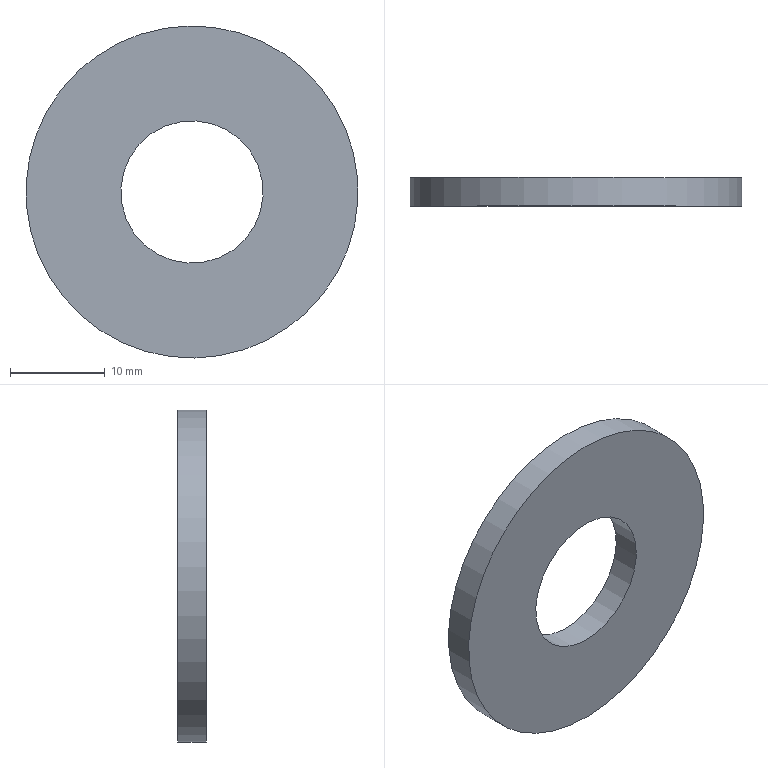Component | NX | RETAINING_RING | 1 solid | 4 faces | box 35 x 3 x 35 mm | volume 2356 mm3 | cylinder 2 | plane 2 | commonest cylinder face diameters 35 x1 15 x1
STEP:
#1=CARTESIAN_POINT('',(0.,0.,0.));
#2=DIRECTION('',(0.,0.,1.));
#3=DIRECTION('',(1.,0.,0.));
#4=AXIS2_PLACEMENT_3D('',#1,#2,#3);
#5=CARTESIAN_POINT('',(646.363,-282.302,-1469.318));
#6=VERTEX_POINT('',#5);
#7=CARTESIAN_POINT('',(630.189,-282.302,-1476.));
#8=DIRECTION('',(0.,-1.,0.));
#9=DIRECTION('',(0.9242,0.,0.3818));
#10=AXIS2_PLACEMENT_3D('',#7,#8,#9);
#11=CIRCLE('',#10,17.5);
#12=CARTESIAN_POINT('',(630.189,-282.302,-1476.));
#13=DIRECTION('',(0.,1.,0.));
#14=DIRECTION('',(-0.9242,0.,-0.3818));
#15=AXIS2_PLACEMENT_3D('',#12,#13,#14);
#16=CYLINDRICAL_SURFACE('',#15,17.5);
#17=CARTESIAN_POINT('',(9.425,0.));
#18=DIRECTION('',(-1.,0.));
#19=VECTOR('',#18,1.);
#20=LINE('',#17,#19);
#21=(GEOMETRIC_REPRESENTATION_CONTEXT(2)PARAMETRIC_REPRESENTATION_CONTEXT()REPRESENTATION_CONTEXT('',''));
#22=DEFINITIONAL_REPRESENTATION('',(#20),#21);
#23=PCURVE('',#16,#22);
#24=CARTESIAN_POINT('',(630.189,-282.302,-1476.));
#25=DIRECTION('',(0.,-1.,0.));
#26=DIRECTION('',(0.9242,0.,0.3818));
#27=AXIS2_PLACEMENT_3D('',#24,#25,#26);
#28=PLANE('',#27);
#29=CARTESIAN_POINT('',(0.,0.));
#30=DIRECTION('',(1.,0.));
#31=AXIS2_PLACEMENT_2D('',#29,#30);
#32=CIRCLE('',#31,17.5);
#33=(GEOMETRIC_REPRESENTATION_CONTEXT(2)PARAMETRIC_REPRESENTATION_CONTEXT()REPRESENTATION_CONTEXT('',''));
#34=DEFINITIONAL_REPRESENTATION('',(#32),#33);
#35=PCURVE('',#28,#34);
#36=SURFACE_CURVE('',#11,(#23,#35),.PCURVE_S1.);
#37=EDGE_CURVE('',#6,#6,#36,.T.);
#38=ORIENTED_EDGE('',*,*,#37,.F.);
#39=CARTESIAN_POINT('',(646.363,-279.302,-1469.318));
#40=VERTEX_POINT('',#39);
#41=CARTESIAN_POINT('',(646.363,-282.302,-1469.318));
#42=CARTESIAN_POINT('',(646.363,-279.302,-1469.318));
#43=B_SPLINE_CURVE_WITH_KNOTS('',1,(#41,#42),.UNSPECIFIED.,.F.,.F.,(2,2),(0.,3.),.PIECEWISE_BEZIER_KNOTS.);
#44=CARTESIAN_POINT('',(9.425,0.));
#45=DIRECTION('',(0.,1.));
#46=VECTOR('',#45,1.);
#47=LINE('',#44,#46);
#48=(GEOMETRIC_REPRESENTATION_CONTEXT(2)PARAMETRIC_REPRESENTATION_CONTEXT()REPRESENTATION_CONTEXT('',''));
#49=DEFINITIONAL_REPRESENTATION('',(#47),#48);
#50=PCURVE('',#16,#49);
#51=CARTESIAN_POINT('',(3.142,0.));
#52=DIRECTION('',(0.,1.));
#53=VECTOR('',#52,1.);
#54=LINE('',#51,#53);
#55=(GEOMETRIC_REPRESENTATION_CONTEXT(2)PARAMETRIC_REPRESENTATION_CONTEXT()REPRESENTATION_CONTEXT('',''));
#56=DEFINITIONAL_REPRESENTATION('',(#54),#55);
#57=PCURVE('',#16,#56);
#58=SEAM_CURVE('',#43,(#50,#57),.PCURVE_S1.);
#59=EDGE_CURVE('',#6,#40,#58,.T.);
#60=ORIENTED_EDGE('',*,*,#59,.T.);
#61=CARTESIAN_POINT('',(630.189,-279.302,-1476.));
#62=DIRECTION('',(0.,-1.,0.));
#63=DIRECTION('',(0.9242,0.,0.3818));
#64=AXIS2_PLACEMENT_3D('',#61,#62,#63);
#65=CIRCLE('',#64,17.5);
#66=CARTESIAN_POINT('',(9.425,3.));
#67=DIRECTION('',(-1.,0.));
#68=VECTOR('',#67,1.);
#69=LINE('',#66,#68);
#70=(GEOMETRIC_REPRESENTATION_CONTEXT(2)PARAMETRIC_REPRESENTATION_CONTEXT()REPRESENTATION_CONTEXT('',''));
#71=DEFINITIONAL_REPRESENTATION('',(#69),#70);
#72=PCURVE('',#16,#71);
#73=CARTESIAN_POINT('',(630.189,-279.302,-1476.));
#74=DIRECTION('',(0.,-1.,0.));
#75=DIRECTION('',(0.9242,0.,0.3818));
#76=AXIS2_PLACEMENT_3D('',#73,#74,#75);
#77=PLANE('',#76);
#78=CARTESIAN_POINT('',(0.,0.));
#79=DIRECTION('',(1.,0.));
#80=AXIS2_PLACEMENT_2D('',#78,#79);
#81=CIRCLE('',#80,17.5);
#82=(GEOMETRIC_REPRESENTATION_CONTEXT(2)PARAMETRIC_REPRESENTATION_CONTEXT()REPRESENTATION_CONTEXT('',''));
#83=DEFINITIONAL_REPRESENTATION('',(#81),#82);
#84=PCURVE('',#77,#83);
#85=SURFACE_CURVE('',#65,(#72,#84),.PCURVE_S1.);
#86=EDGE_CURVE('',#40,#40,#85,.T.);
#87=ORIENTED_EDGE('',*,*,#86,.T.);
#88=ORIENTED_EDGE('',*,*,#59,.F.);
#89=EDGE_LOOP('',(#38,#60,#87,#88));
#90=FACE_BOUND('',#89,.T.);
#91=ADVANCED_FACE('',(#90),#16,.T.);
#92=CARTESIAN_POINT('',(637.121,-282.302,-1473.136));
#93=VERTEX_POINT('',#92);
#94=CARTESIAN_POINT('',(630.189,-282.302,-1476.));
#95=DIRECTION('',(0.,-1.,0.));
#96=DIRECTION('',(0.9242,0.,0.3818));
#97=AXIS2_PLACEMENT_3D('',#94,#95,#96);
#98=CIRCLE('',#97,7.5);
#99=CARTESIAN_POINT('',(630.189,-282.302,-1476.));
#100=DIRECTION('',(0.,1.,0.));
#101=DIRECTION('',(-0.9242,0.,-0.3818));
#102=AXIS2_PLACEMENT_3D('',#99,#100,#101);
#103=CYLINDRICAL_SURFACE('',#102,7.5);
#104=CARTESIAN_POINT('',(9.425,0.));
#105=DIRECTION('',(-1.,0.));
#106=VECTOR('',#105,1.);
#107=LINE('',#104,#106);
#108=(GEOMETRIC_REPRESENTATION_CONTEXT(2)PARAMETRIC_REPRESENTATION_CONTEXT()REPRESENTATION_CONTEXT('',''));
#109=DEFINITIONAL_REPRESENTATION('',(#107),#108);
#110=PCURVE('',#103,#109);
#111=CARTESIAN_POINT('',(0.,0.));
#112=DIRECTION('',(1.,0.));
#113=AXIS2_PLACEMENT_2D('',#111,#112);
#114=CIRCLE('',#113,7.5);
#115=(GEOMETRIC_REPRESENTATION_CONTEXT(2)PARAMETRIC_REPRESENTATION_CONTEXT()REPRESENTATION_CONTEXT('',''));
#116=DEFINITIONAL_REPRESENTATION('',(#114),#115);
#117=PCURVE('',#28,#116);
#118=SURFACE_CURVE('',#98,(#110,#117),.PCURVE_S1.);
#119=EDGE_CURVE('',#93,#93,#118,.T.);
#120=ORIENTED_EDGE('',*,*,#119,.F.);
#121=CARTESIAN_POINT('',(637.121,-279.302,-1473.136));
#122=VERTEX_POINT('',#121);
#123=CARTESIAN_POINT('',(637.121,-282.302,-1473.136));
#124=CARTESIAN_POINT('',(637.121,-279.302,-1473.136));
#125=B_SPLINE_CURVE_WITH_KNOTS('',1,(#123,#124),.UNSPECIFIED.,.F.,.F.,(2,2),(0.,3.),.PIECEWISE_BEZIER_KNOTS.);
#126=CARTESIAN_POINT('',(9.425,0.));
#127=DIRECTION('',(0.,1.));
#128=VECTOR('',#127,1.);
#129=LINE('',#126,#128);
#130=(GEOMETRIC_REPRESENTATION_CONTEXT(2)PARAMETRIC_REPRESENTATION_CONTEXT()REPRESENTATION_CONTEXT('',''));
#131=DEFINITIONAL_REPRESENTATION('',(#129),#130);
#132=PCURVE('',#103,#131);
#133=CARTESIAN_POINT('',(3.142,0.));
#134=DIRECTION('',(0.,1.));
#135=VECTOR('',#134,1.);
#136=LINE('',#133,#135);
#137=(GEOMETRIC_REPRESENTATION_CONTEXT(2)PARAMETRIC_REPRESENTATION_CONTEXT()REPRESENTATION_CONTEXT('',''));
#138=DEFINITIONAL_REPRESENTATION('',(#136),#137);
#139=PCURVE('',#103,#138);
#140=SEAM_CURVE('',#125,(#132,#139),.PCURVE_S1.);
#141=EDGE_CURVE('',#93,#122,#140,.T.);
#142=ORIENTED_EDGE('',*,*,#141,.T.);
#143=CARTESIAN_POINT('',(630.189,-279.302,-1476.));
#144=DIRECTION('',(0.,-1.,0.));
#145=DIRECTION('',(0.9242,0.,0.3818));
#146=AXIS2_PLACEMENT_3D('',#143,#144,#145);
#147=CIRCLE('',#146,7.5);
#148=CARTESIAN_POINT('',(9.425,3.));
#149=DIRECTION('',(-1.,0.));
#150=VECTOR('',#149,1.);
#151=LINE('',#148,#150);
#152=(GEOMETRIC_REPRESENTATION_CONTEXT(2)PARAMETRIC_REPRESENTATION_CONTEXT()REPRESENTATION_CONTEXT('',''));
#153=DEFINITIONAL_REPRESENTATION('',(#151),#152);
#154=PCURVE('',#103,#153);
#155=CARTESIAN_POINT('',(0.,0.));
#156=DIRECTION('',(1.,0.));
#157=AXIS2_PLACEMENT_2D('',#155,#156);
#158=CIRCLE('',#157,7.5);
#159=(GEOMETRIC_REPRESENTATION_CONTEXT(2)PARAMETRIC_REPRESENTATION_CONTEXT()REPRESENTATION_CONTEXT('',''));
#160=DEFINITIONAL_REPRESENTATION('',(#158),#159);
#161=PCURVE('',#77,#160);
#162=SURFACE_CURVE('',#147,(#154,#161),.PCURVE_S1.);
#163=EDGE_CURVE('',#122,#122,#162,.T.);
#164=ORIENTED_EDGE('',*,*,#163,.T.);
#165=ORIENTED_EDGE('',*,*,#141,.F.);
#166=EDGE_LOOP('',(#120,#142,#164,#165));
#167=FACE_BOUND('',#166,.F.);
#168=ADVANCED_FACE('',(#167),#103,.F.);
#169=ORIENTED_EDGE('',*,*,#37,.T.);
#170=EDGE_LOOP('',(#169));
#171=FACE_BOUND('',#170,.T.);
#172=ORIENTED_EDGE('',*,*,#119,.F.);
#173=EDGE_LOOP('',(#172));
#174=FACE_BOUND('',#173,.T.);
#175=ADVANCED_FACE('',(#171,#174),#28,.T.);
#176=ORIENTED_EDGE('',*,*,#86,.F.);
#177=EDGE_LOOP('',(#176));
#178=FACE_BOUND('',#177,.T.);
#179=ORIENTED_EDGE('',*,*,#163,.T.);
#180=EDGE_LOOP('',(#179));
#181=FACE_BOUND('',#180,.T.);
#182=ADVANCED_FACE('',(#178,#181),#77,.F.);
#183=CLOSED_SHELL('',(#91,#168,#175,#182));
#184=MANIFOLD_SOLID_BREP('',#183);
#185=(LENGTH_UNIT()NAMED_UNIT(*)SI_UNIT(.MILLI.,.METRE.));
#186=UNCERTAINTY_MEASURE_WITH_UNIT(LENGTH_MEASURE(0.00001),#185,'','');
#187=(NAMED_UNIT(*)PLANE_ANGLE_UNIT()SI_UNIT($,.RADIAN.));
#188=(NAMED_UNIT(*)SI_UNIT($,.STERADIAN.)SOLID_ANGLE_UNIT());
#189=(GEOMETRIC_REPRESENTATION_CONTEXT(3)GLOBAL_UNCERTAINTY_ASSIGNED_CONTEXT((#186))GLOBAL_UNIT_ASSIGNED_CONTEXT((#185,#187,#188))REPRESENTATION_CONTEXT('',''));
#190=ADVANCED_BREP_SHAPE_REPRESENTATION('',(#4,#184),#189);